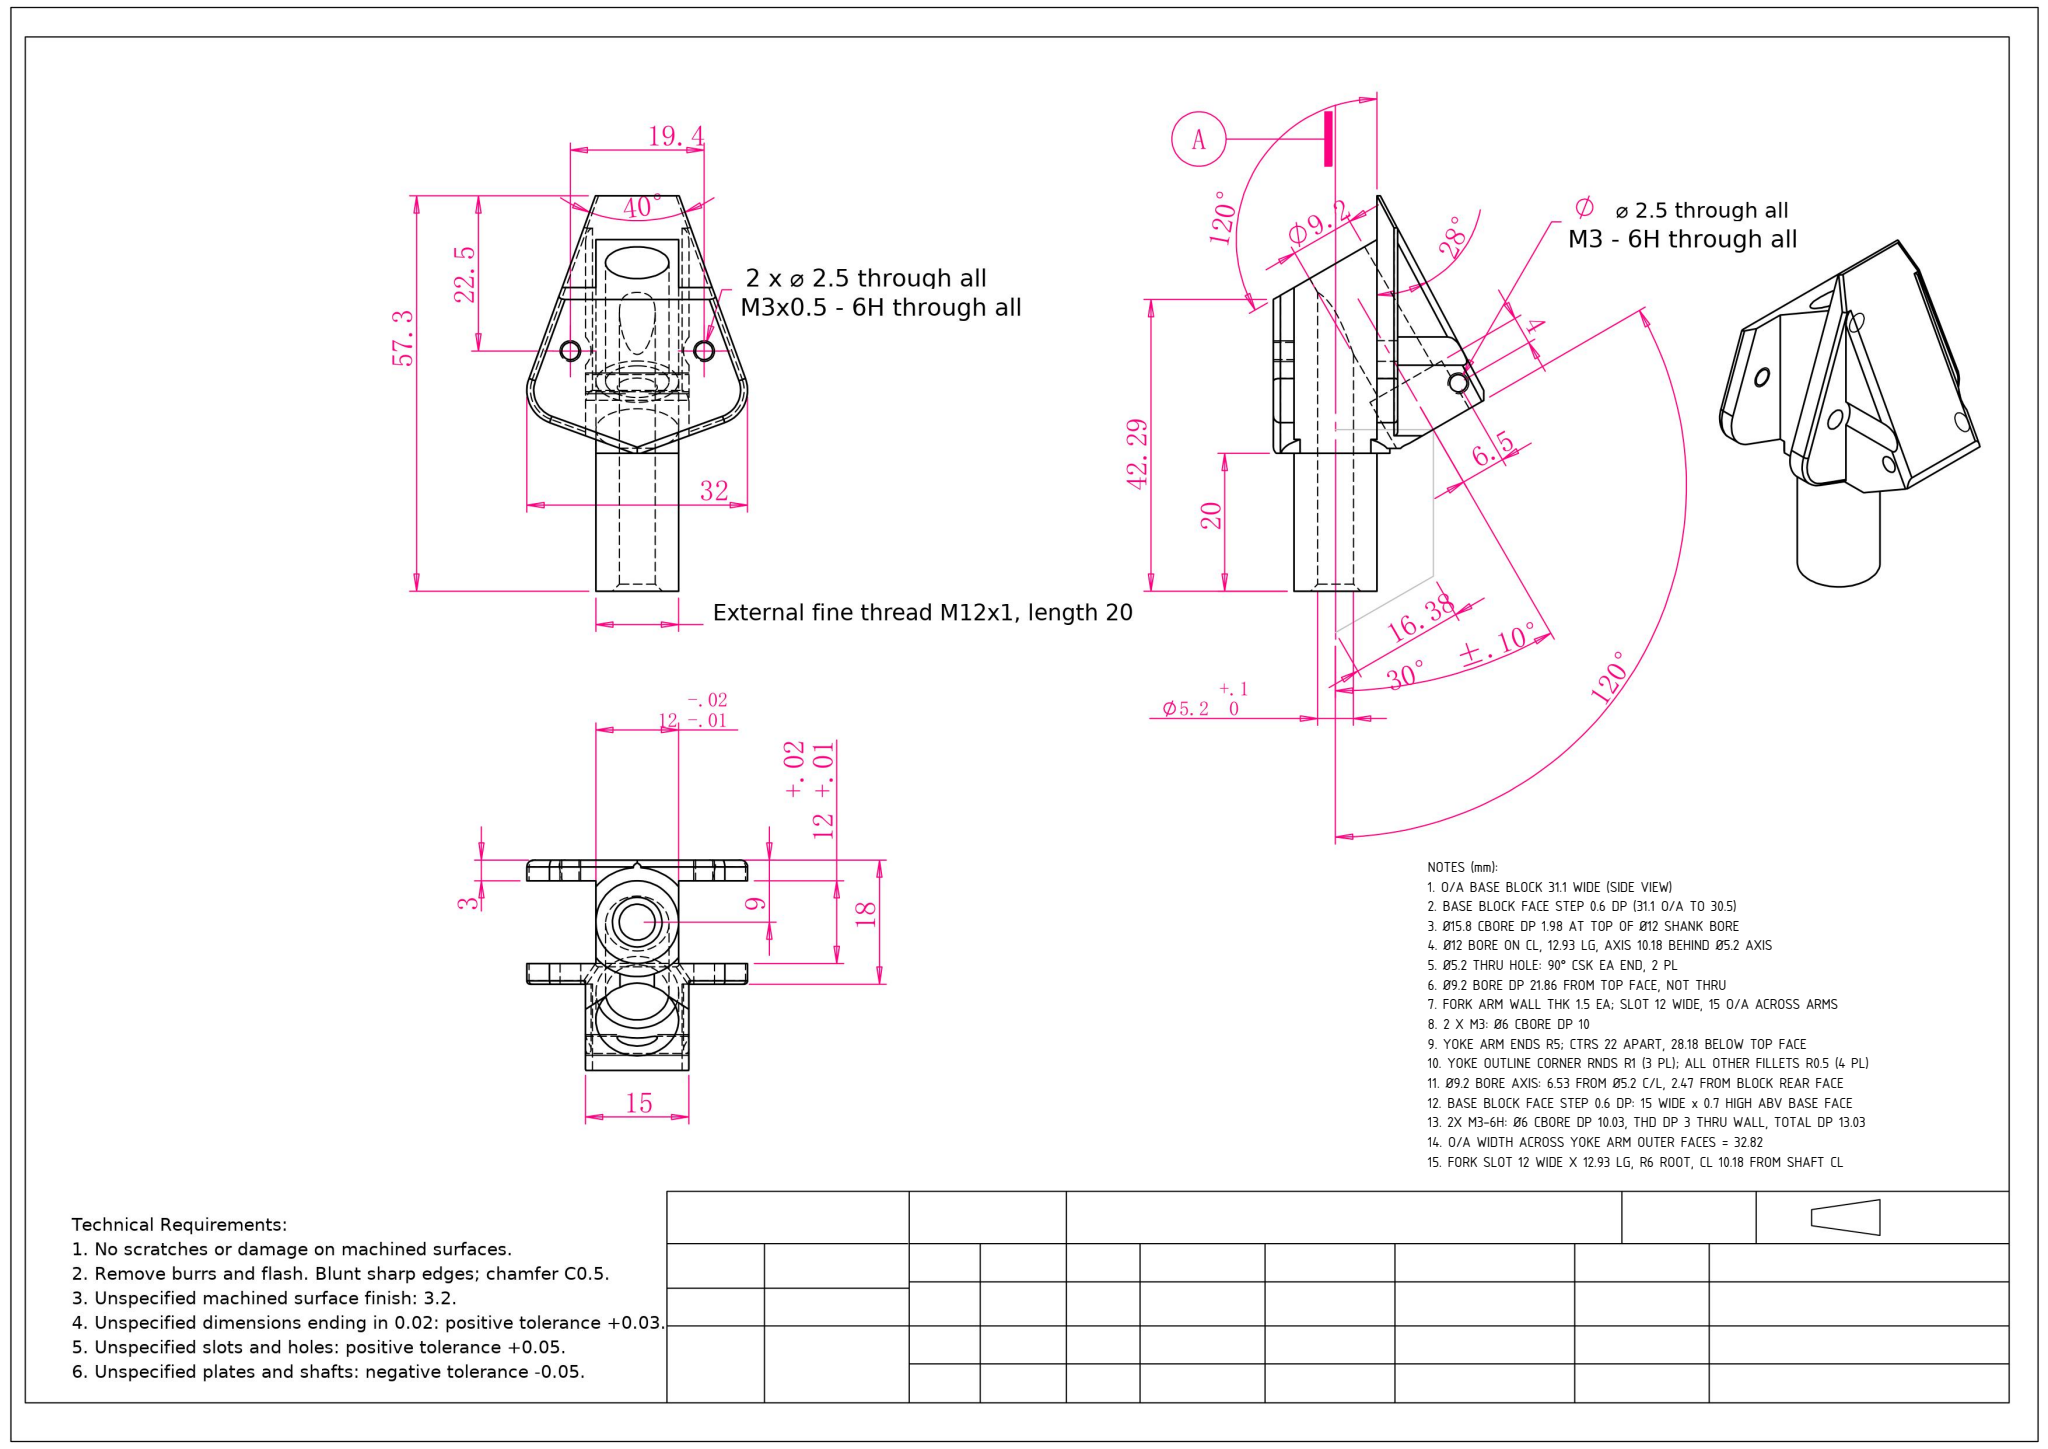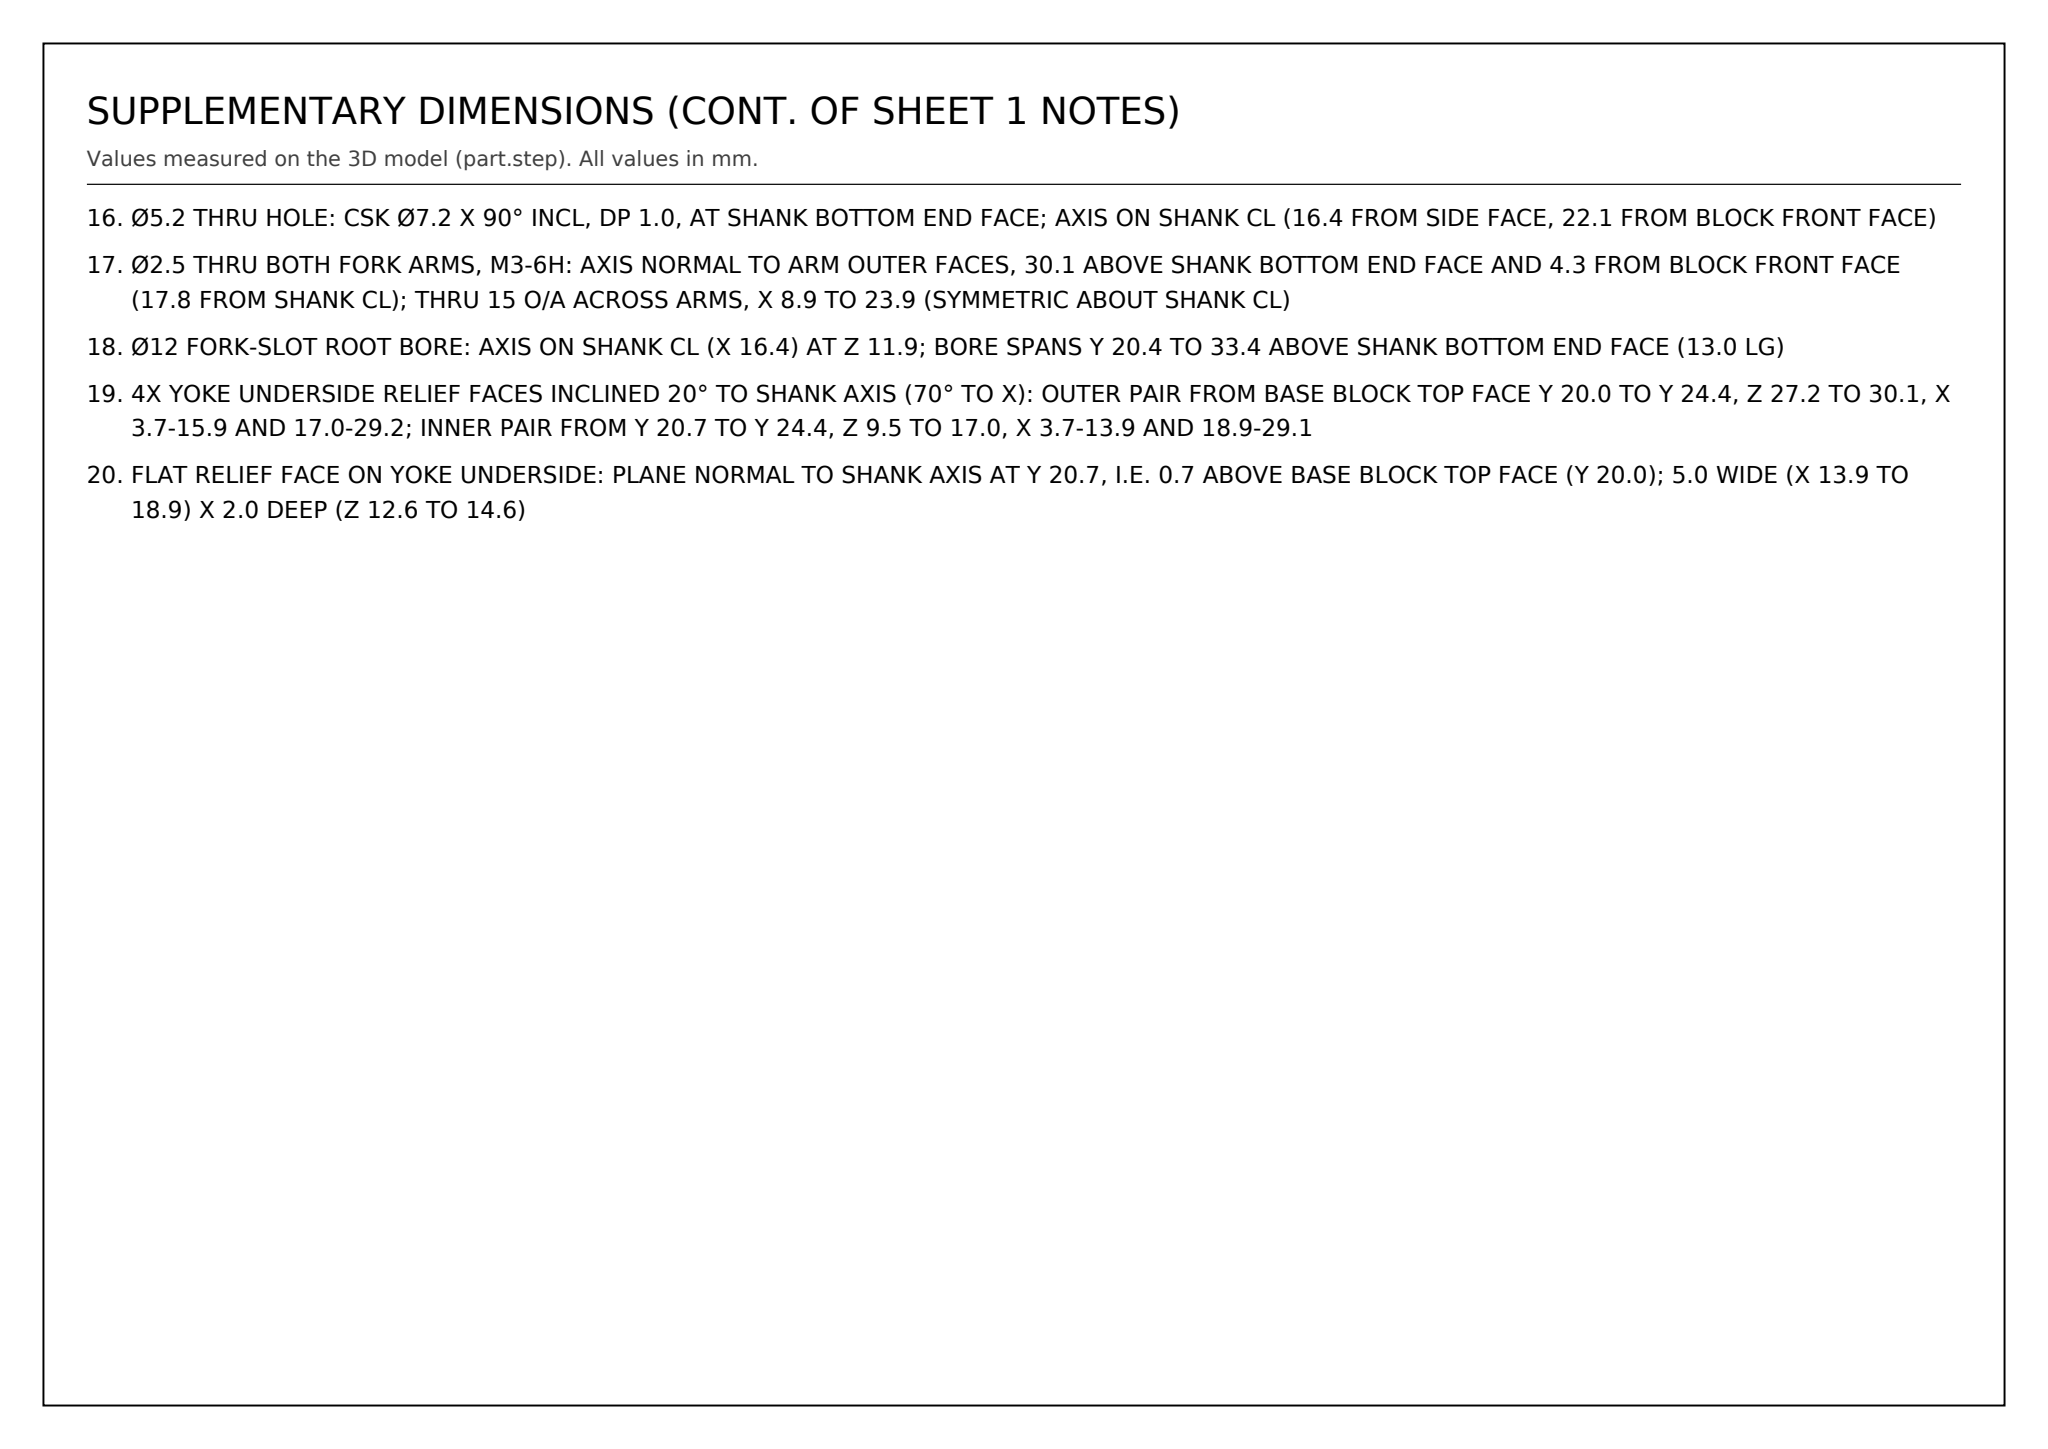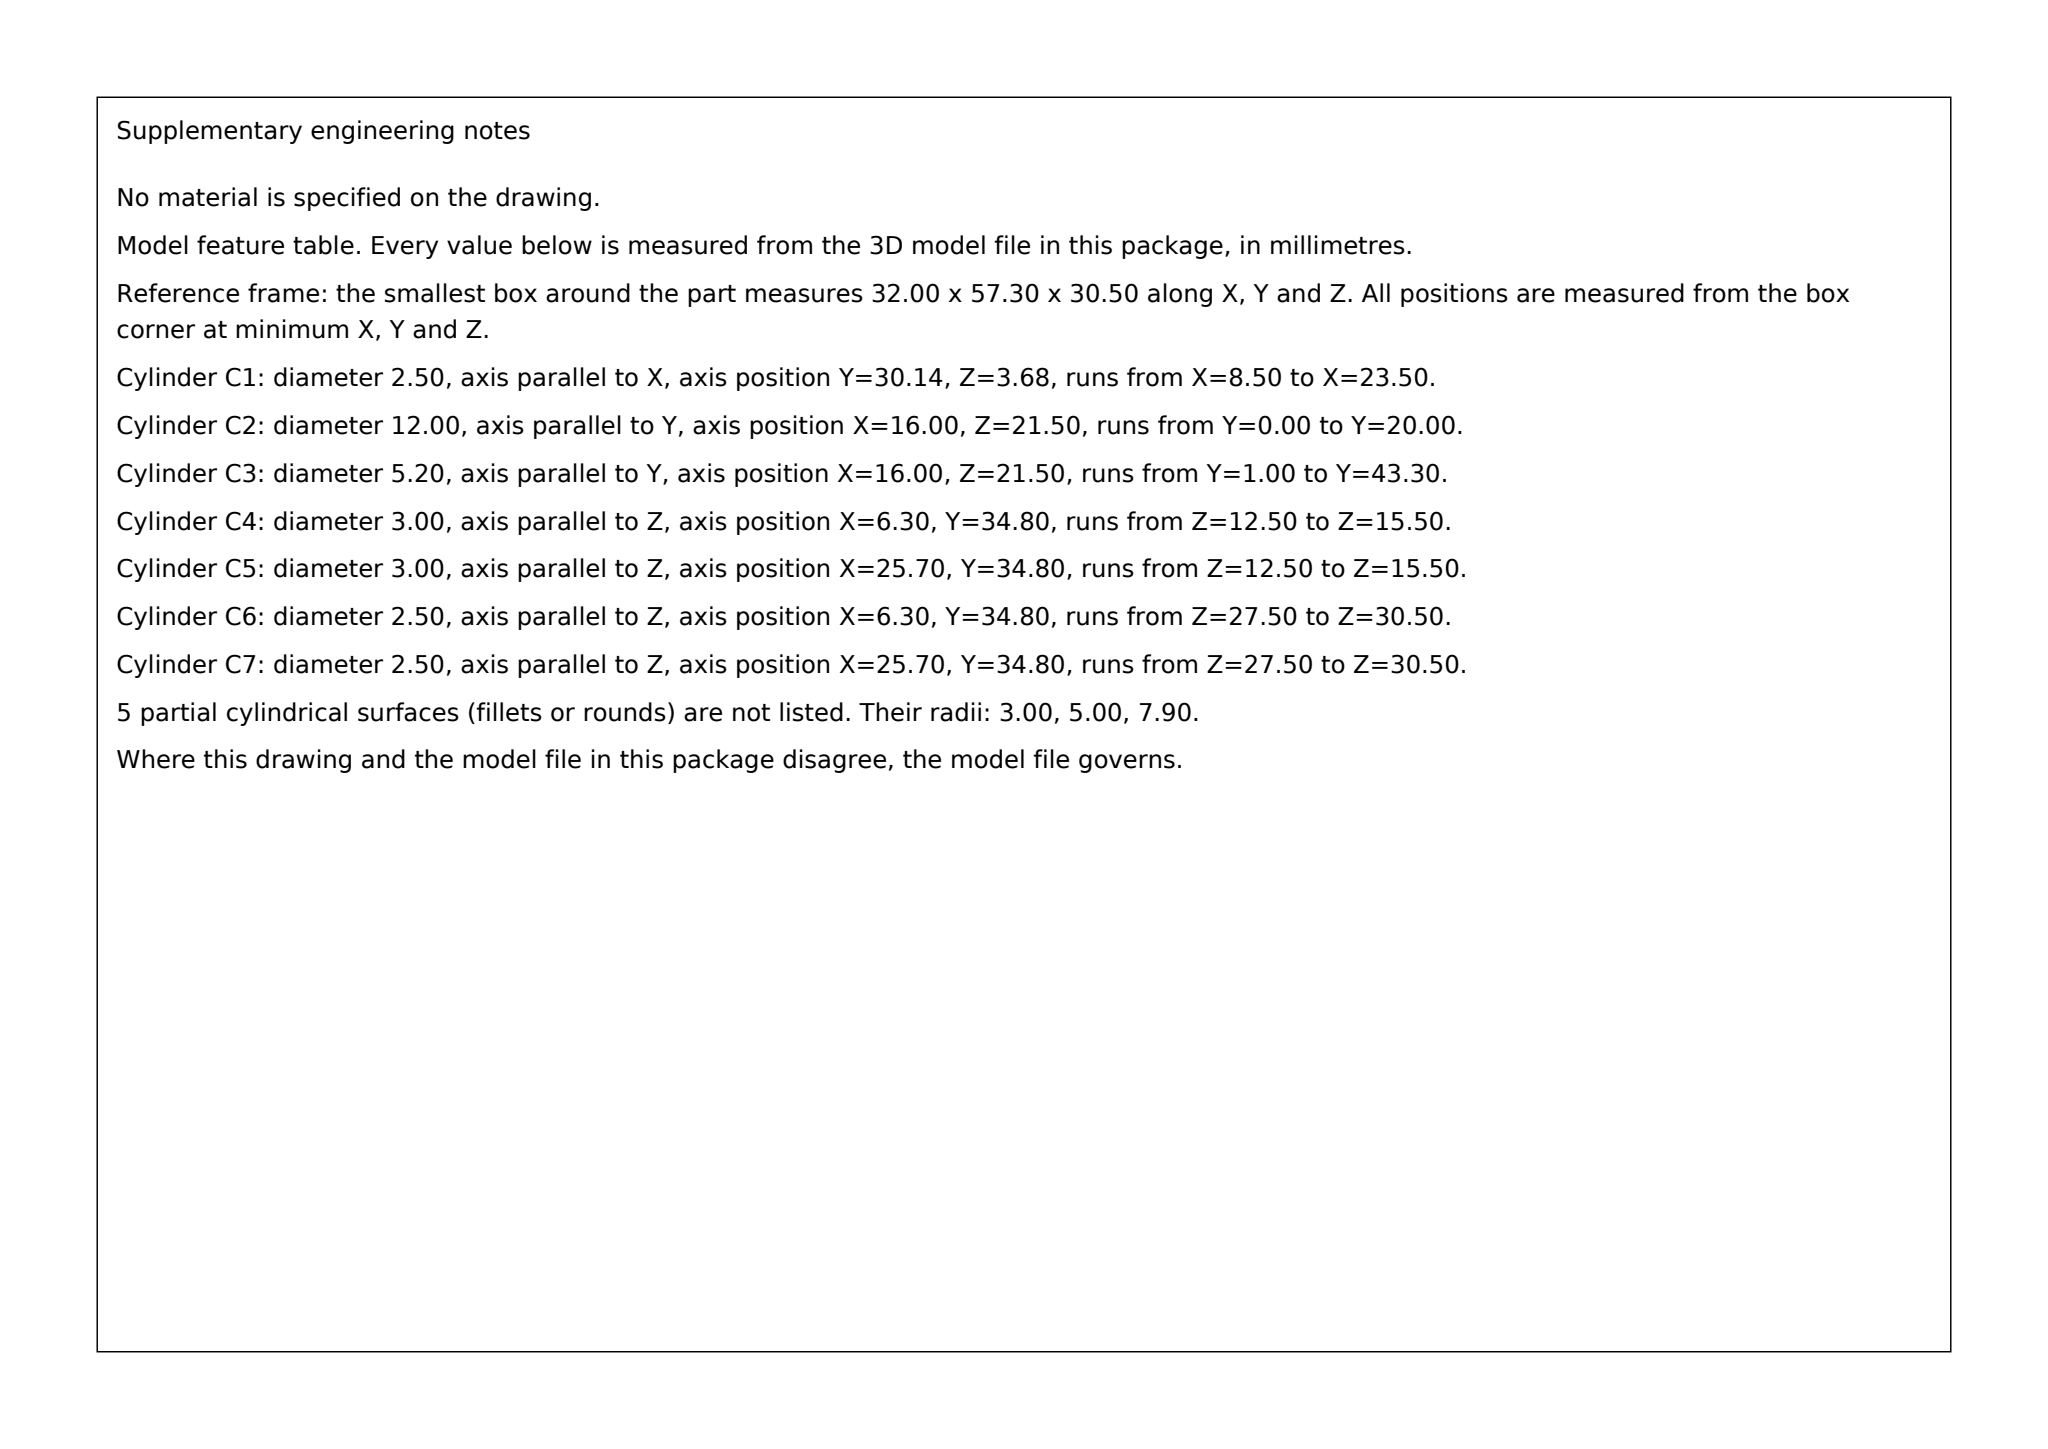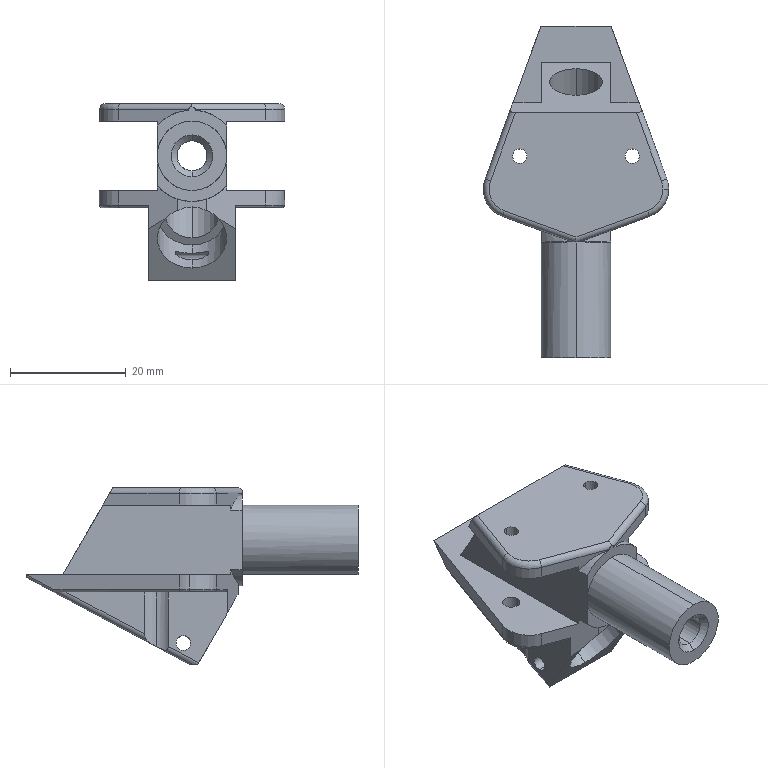Part | SolidWorks | mm | 1 solid | 82 faces | box 32 x 57.3 x 30.5 mm | volume 10257 mm3 | cylinder 43 | plane 30 | torus 7 | cone 2 | commonest cylinder face diameters 2.5 x6 10 x6 2 x6 1 x6 12 x4 3 x4 15.8 x4 6 x3
Drawing notes:
O/A BASE BLOCK 31.1 WIDE (SIDE VIEW) | from the solid: bbox_xyz z = 31.101; z planes 0.6 ... 31.1
BASE BLOCK FACE STEP 0.6 DP (31.1 O/A TO 30.5) | from the solid: z-plane at 0.6 vs bbox z 0...31.101; 31.1-0.6=30.5
Ø15.8 CBORE DP 1.98 AT TOP OF Ø12 SHANK BORE | from the solid: Ø15.8 cyl axis y at (x16.41,z22.1) L=1.98, coaxial with Ø12 (L=20) shank
Ø12 BORE ON CL, 12.93 LG, AXIS 10.18 BEHIND Ø5.2 AXIS | from the solid: cyl dia12 axis y at (x16.41,z11.92) L=12.93; 22.10-11.92=10.18; x16.41 = CL
Ø5.2 THRU HOLE: 90° CSK EA END, 2 PL | from the solid: cones [90.0, 5.2] count 2 on Ø5.2 y-axis hole (len 42.3)
Ø9.2 BORE DP 21.86 FROM TOP FACE, NOT THRU | from the solid: cyl [9.2, axis y, (16.41, 28.63), L=21.86]; top plane y=57.3 -> ends y=35.44
FORK ARM WALL THK 1.5 EA; SLOT 12 WIDE, 15 O/A ACROSS ARMS | from the solid: x planes 8.91 & 10.41, 22.41 & 23.91 -> 1.5 thk; 10.41-22.41=12; 23.91-8.91=15
2 X M3: Ø6 CBORE DP 10 | from the solid: Ø6 cyls axis z at (6.71,34.8) & (26.11,34.8), L=10.03 (9.44 cut by face)
YOKE ARM ENDS R5; CTRS 22 APART, 28.18 BELOW TOP FACE | from the solid: Ø10 cyls axis z at (5.41,29.12) & (27.41,29.12); 27.41-5.41=22; 57.3-29.12=28.18
YOKE OUTLINE CORNER RNDS R1 (3 PL); ALL OTHER FILLETS R0.5 (4 PL) | from the solid: fillet_radii: [1.0, 3] on triangular-outline corners; [0.5, 4] remaining edges
Ø9.2 BORE AXIS: 6.53 FROM Ø5.2 C/L, 2.47 FROM BLOCK REAR FACE | from the solid: Ø9.2 y-axis cyl at (x16.41,z28.63); Ø5.2 y-axis cyl at (x16.41,z22.10) -> 6.53 offset; z plane 31.1 rear face -> 2.47
BASE BLOCK FACE STEP 0.6 DP: 15 WIDE x 0.7 HIGH ABV BASE FACE | from the solid: z plane 0.6 (step face); x planes 8.91 & 23.91 -> 15 wide, symm about C/L x16.41; y planes 20.0 (base face) & 20.7 -> 0.7 high
2X M3-6H: Ø6 CBORE DP 10.03, THD DP 3 THRU WALL, TOTAL DP 13.03 | from the solid: Ø6 z-cyl at (6.71,34.8) & (26.11,34.8) L=10.03 (one split seg 9.44); Ø2.5/Ø3 z-cyl same axes L=3.0; wall planes z=28.1 to z=31.1 = 3 THK
O/A WIDTH ACROSS YOKE ARM OUTER FACES = 32.82 | from the solid: bbox_xyz x = 32.824 (vs x-planes 8.91/23.91 = 15 O/A across fork arms)
FORK SLOT 12 WIDE X 12.93 LG, R6 ROOT, CL 10.18 FROM SHAFT CL | from the solid: x-planes 10.41/22.41 = 12 slot; Ø12 y-cyl at (x16.41,z11.92) L=12.93 is slot root (R6); M12 shaft/Ø5.2 axis at z=22.1 -> 22.1-11.92=10.18
Ø5.2 THRU HOLE: CSK Ø7.2 X 90° INCL, DP 1.0, AT SHANK BOTTOM END FACE; AXIS ON SHANK CL (16.4 FROM SIDE FACE, 22.1 FROM BLOCK FRONT FACE) | from the solid: cones[90.0, ref_dia 5.2, bbox_from [12.8,0.0,18.5] / [16.4,0.0,18.5], size [3.6,1.0,7.2]] with hole/bore Ø5.2 axis y at [16.4,-,22.1] from y0.0 (1.0) to 43.3
Ø2.5 THRU BOTH FORK ARMS, M3-6H: AXIS NORMAL TO ARM OUTER FACES, 30.1 ABOVE SHANK BOTTOM END FACE AND 4.3 FROM BLOCK FRONT FACE (17.8 FROM SHANK CL); THRU 15 O/A ACROSS ARMS, X 8.9 TO 23.9 (SYMMETRIC ABOUT SHANK CL) | from the solid: cylinders hole/bore Ø2.5 axis x, axis_pos [y 30.1, z 4.3], from 8.9 to 23.9; shank Ø12 axis y at [16.4,-,22.1]
Ø12 FORK-SLOT ROOT BORE: AXIS ON SHANK CL (X 16.4) AT Z 11.9; BORE SPANS Y 20.4 TO 33.4 ABOVE SHANK BOTTOM END FACE (13.0 LG) | from the solid: cylinders: hole/bore dia 12.0 inclined, axis_pos [16.4,null,11.9], from 20.4 to 33.4
4X YOKE UNDERSIDE RELIEF FACES INCLINED 20° TO SHANK AXIS (70° TO X): OUTER PAIR FROM BASE BLOCK TOP FACE Y 20.0 TO Y 24.4, Z 27.2 TO 30.1, X 3.7-15.9 AND 17.0-29.2; INNER PAIR FROM Y 20.7 TO Y 24.4, Z 9.5 TO 17.0, X 3.7-13.9 AND 18.9-29.1 | from the solid: inclined_planes angle_to_xyz [70,20,90] x4 at bbox_from [17.0,20.0,27.2], [3.7,20.0,27.2], [18.9,20.7,9.5], [3.7,20.7,9.5]
FLAT RELIEF FACE ON YOKE UNDERSIDE: PLANE NORMAL TO SHANK AXIS AT Y 20.7, I.E. 0.7 ABOVE BASE BLOCK TOP FACE (Y 20.0); 5.0 WIDE (X 13.9 TO 18.9) X 2.0 DEEP (Z 12.6 TO 14.6) | from the solid: axis_planes: ['y',20.7, extent {'x':[13.9,18.9],'z':[12.6,14.6]}, area 6]
build123d program:
from build123d import *

# Parameters (mm, degrees)
SKETCH1_R                    = 10
EXTRUDE1_DEPTH               = 18.8
SKETCH2_R                    = 7.9
EXTRUDE2_DEPTH               = 37
EXTRUDE3_DEPTH               = 3.5
CUT_EXTRUDE1_DEPTH           = 2.5
CUT_EXTRUDE2_DEPTH           = 50
EXTRUDE5_DEPTH               = 14
CUT_EXTRUDE3_DEPTH           = 12.5
CUT_EXTRUDE4_DEPTH           = 50
CUT_EXTRUDE5_DEPTH           = 50
EXTRUDE9_DEPTH               = 0.5
CUT_EXTRUDE18_DEPTH          = 250
FILLET15_R                   = 1
FILLET16_R                   = 1
FILLET17_R                   = 1
SKETCH11_R                   = 1.2
CUT_EXTRUDE7_DEPTH           = 5
F_3_0_3_DIAMETER_HOLE1_D     = 3
F_3_0_3_DIAMETER_HOLE1_DEPTH = 8.5
SKETCH14_R                   = 2.6
CUT_EXTRUDE8_DEPTH           = 69.74
M16_TAPPED_HOLE1_D           = 14
M16_TAPPED_HOLE1_DEPTH       = 13
M16_TAPPED_HOLE1_TIP         = 4.206
EXTRUDE10_REACH              = 70.74
SKETCH52_R                   = 2.6
SKETCH52_R_2                 = 2.55
CUT_EXTRUDE9_REACH           = 60.671
SKETCH17_R                   = 4.6
SKETCH18_R                   = 6
CUT_EXTRUDE10_DEPTH          = 8
EXTRUDE8_REACH               = 70.74
SKETCH30_R                   = 7
SKETCH30_R_2                 = 2.55
SKETCH31_OUTSIDE_W           = 49.522
SKETCH31_OUTSIDE_H           = 49.022
SKETCH31_OUTSIDE_R           = 6
CUT_EXTRUDE17_DEPTH          = 26
CHAMFER1_SIZE                = 1
CUT_EXTRUDE19_DEPTH          = 71.379
CUT_EXTRUDE20_DEPTH          = 71.379
CUT_EXTRUDE21_DEPTH          = 71.379
M3_TAPPED_HOLE5_D            = 2.5
M3_TAPPED_HOLE6_D            = 2.5
SKETCH50_R                   = 3
SKETCH50_R_2                 = 3
CUT_EXTRUDE23_DEPTH          = 68.727
FILLET18_R                   = 0.5
SKETCH53_R                   = 6
CUT_EXTRUDE24_DEPTH          = 6
SKETCH54_R                   = 2.6
CUT_EXTRUDE25_DEPTH          = 64.258
CHAMFER2_SIZE                = 1


with BuildPart() as part:
    # Sketch1 → Extrude1 (new body)
    with BuildSketch(Plane(origin=(0, 0, 0), x_dir=(1, 0, 0), z_dir=(0, 1, 0))):
        with Locations(Location((0, 0, 0), (0, 0, 270))):
            Circle(SKETCH1_R)
    extrude(amount=EXTRUDE1_DEPTH)

    # Sketch2 → Extrude2 (add)
    with BuildSketch(Plane(origin=(0, 18.8, 0), x_dir=(-1, 0, 0), z_dir=(0, 1, 0))):
        with Locations(Location((0, 0, 0), (0, 0, 90))):
            Circle(SKETCH2_R)
    extrude(amount=EXTRUDE2_DEPTH)

    # Sketch3 → Extrude3 (add)
    with BuildSketch(Plane.XY.offset(8.5)):
        with BuildLine():
            Line((0, 25.8), (12.71, 30.426))
            ThreePointArc((12.71, 30.426), (15.532, 33.011), (15.698, 36.835))
            Line((15.698, 36.835), (6.066, 63.3))
            Line((6.066, 63.3), (-6.066, 63.3))
            Line((-6.066, 63.3), (-15.698, 36.835))
            ThreePointArc((-15.698, 36.835), (-15.532, 33.011), (-12.71, 30.426))
            Line((-12.71, 30.426), (0, 25.8))
        make_face()
    extrude3 = extrude(amount=-EXTRUDE3_DEPTH)

    # Mirror1: Extrude3 across plane
    add(extrude3.mirror(Plane.XY.offset(0.5)))

    # Sketch4 → Cut-Extrude1 (cut)
    with BuildSketch(Plane(origin=(8.5, 0, 0), x_dir=(0, 0, -1), z_dir=(1, 0, 0))):
        with BuildLine():
            Line((4, 36.835), (4, 63.3))
            Line((4, 63.3), (-5, 63.3))
            Line((-5, 63.3), (-5, 36.835))
            Line((-5, 36.835), (-5, 26.3))
            ThreePointArc((-5, 26.3), (-0.5, 21.8), (4, 26.3))
            Line((4, 26.3), (4, 36.835))
        make_face()
    cut_extrude1 = extrude(amount=-CUT_EXTRUDE1_DEPTH, mode=Mode.SUBTRACT)

    # Mirror2: Cut-Extrude1 across plane
    add(cut_extrude1.mirror(Plane(origin=(0, 0, 0), x_dir=(0, 0, 1), z_dir=(1, 0, 0))), mode=Mode.SUBTRACT)

    # Sketch5 → Cut-Extrude2 (cut, symmetric)
    with BuildSketch(Plane(origin=(0, 0, 0), x_dir=(0, 0, -1), z_dir=(1, 0, 0))):
        Polygon((4, 55.8), (-8.5, 48.583), (-8.5, 63.3), (4, 63.3), align=None)
    extrude(amount=CUT_EXTRUDE2_DEPTH, both=True, mode=Mode.SUBTRACT)

    # Sketch6 → Extrude5 (add)
    with BuildSketch(Plane(origin=(0, 0, -7.5), x_dir=(-1, 0, 0), z_dir=(0, 0, -1))):
        with BuildLine():
            Line((-2.482, 26.703), (2.482, 26.703))
            Line((2.482, 26.703), (12.71, 30.426))
            ThreePointArc((12.71, 30.426), (15.532, 33.011), (15.698, 36.835))
            Line((15.698, 36.835), (6.066, 63.3))
            Line((6.066, 63.3), (-6.066, 63.3))
            Line((-6.066, 63.3), (-15.698, 36.835))
            ThreePointArc((-15.698, 36.835), (-15.532, 33.011), (-12.71, 30.426))
            Line((-12.71, 30.426), (-2.482, 26.703))
        make_face()
    extrude(amount=EXTRUDE5_DEPTH)

    # Sketch7 → Cut-Extrude3 (cut)
    with BuildSketch(Plane(origin=(0, 0, -21.5), x_dir=(-1, 0, 0), z_dir=(0, 0, -1))):
        with BuildLine():
            Line((-19.5, 21.015), (-10.465, 23.436))
            ThreePointArc((-10.465, 23.436), (-8.327, 24.865), (-7.5, 27.3))
            Line((-7.5, 27.3), (-7.5, 63.3))
            Line((-7.5, 63.3), (-19.5, 63.3))
            Line((-19.5, 63.3), (-19.5, 21.015))
        make_face()
        with BuildLine():
            Line((19.5, 63.3), (19.5, 21.015))
            Line((19.5, 21.015), (10.465, 23.436))
            ThreePointArc((10.465, 23.436), (8.327, 24.865), (7.5, 27.3))
            Line((7.5, 27.3), (7.5, 63.3))
            Line((7.5, 63.3), (19.5, 63.3))
        make_face()
    extrude(amount=-CUT_EXTRUDE3_DEPTH, mode=Mode.SUBTRACT)

    # Sketch8 → Cut-Extrude4 (cut, symmetric)
    with BuildSketch(Plane(origin=(0, 0, 0), x_dir=(0, 0, -1), z_dir=(1, 0, 0))):
        Polygon((7.9, 25.8), (21.5, 33.652), (21.5, 25.8), align=None)
    extrude(amount=CUT_EXTRUDE4_DEPTH, both=True, mode=Mode.SUBTRACT)

    # Sketch9 → Cut-Extrude5 (cut, symmetric)
    with BuildSketch(Plane(origin=(0, 0, 0), x_dir=(0, 0, -1), z_dir=(1, 0, 0))):
        Polygon((6.5, 63.3), (21.5, 35.089), (21.5, 63.3), align=None)
    extrude(amount=CUT_EXTRUDE5_DEPTH, both=True, mode=Mode.SUBTRACT)

    # Sketch32 → Extrude9 (add)
    with BuildSketch(Plane.XY.offset(8.5)):
        with BuildLine():
            Line((0, 25.8), (12.71, 30.426))
            ThreePointArc((12.71, 30.426), (15.532, 33.011), (15.698, 36.835))
            Line((15.698, 36.835), (11.422, 48.583))
            Line((11.422, 48.583), (-11.422, 48.583))
            Line((-11.422, 48.583), (-15.698, 36.835))
            ThreePointArc((-15.698, 36.835), (-15.532, 33.011), (-12.71, 30.426))
            Line((-12.71, 30.426), (0, 25.8))
        make_face()
    extrude(amount=EXTRUDE9_DEPTH)

    # Sketch34 → Cut-Extrude18 (cut, symmetric)
    with BuildSketch(Plane.ZY.offset(6)):
        Polygon((5, 50.604), (9, 48.294), (9.125, 48.511), (5.125, 50.82), align=None)
    extrude(amount=CUT_EXTRUDE18_DEPTH, both=True, mode=Mode.SUBTRACT)

    # Fillet15
    fillet15_edges = [part.edges().sort_by_distance(p)[0] for p in [
        (-7.5, 46.844, -15.25),
    ]]
    fillet(fillet15_edges, radius=FILLET15_R)

    # Fillet16
    fillet16_edges = [part.edges().sort_by_distance(p)[0] for p in [
        (7.5, 46.844, -15.25),
    ]]
    fillet(fillet16_edges, radius=FILLET16_R)

    # Fillet17
    fillet17_edges = [part.edges().sort_by_distance(p)[0] for p in [
        (-15.532, 33.011, 9),
        (-6.355, 28.113, 9),
        (6.355, 28.113, 9),
        (15.532, 33.011, 9),
        (13.613, 42.565, 9),
        (-13.613, 42.565, 9),
    ]]
    fillet(fillet17_edges, radius=FILLET17_R)

    # Sketch11 → Cut-Extrude7 (cut)
    with BuildSketch(Plane.XY.offset(9)):
        with Locations((-9.7, 40.8)):
            Circle(SKETCH11_R)
        with Locations((9.7, 40.8)):
            Circle(SKETCH11_R)
    extrude(amount=-CUT_EXTRUDE7_DEPTH, mode=Mode.SUBTRACT)

    # 3.0 _3_ Diameter Hole1
    with Locations(Plane.XY.offset(-4)):
        with Locations((-9.7, 40.8), (9.7, 40.8)):
            Hole(F_3_0_3_DIAMETER_HOLE1_D / 2, depth=F_3_0_3_DIAMETER_HOLE1_DEPTH)

    # Sketch14 → Cut-Extrude8 (cut, through all)
    with BuildSketch(Plane.XZ):
        with Locations(Location((0, 0, 0), (0, 0, 270))):
            Circle(SKETCH14_R)
    extrude(amount=-CUT_EXTRUDE8_DEPTH, mode=Mode.SUBTRACT)

    # M16 Tapped Hole1
    with Locations(Plane.XZ):
        with Locations((0, 0)):
            Hole(M16_TAPPED_HOLE1_D / 2, depth=M16_TAPPED_HOLE1_DEPTH)
            with Locations((0, 0, -(M16_TAPPED_HOLE1_DEPTH + M16_TAPPED_HOLE1_TIP / 2))):  # 118° drill point
                Cone(0, M16_TAPPED_HOLE1_D / 2, M16_TAPPED_HOLE1_TIP, mode=Mode.SUBTRACT)

    # Extrude10: up to this plane
    extrude10_end = Plane(origin=(-50, 55.8, -4), z_dir=(0, -0.866, -0.5))
    # Sketch52 → Extrude10 (add, up to the surface)
    with BuildSketch(Plane.XZ, mode=Mode.PRIVATE) as extrude10_sk1:
        with Locations(Location((0, 0, 0), (0, 0, 270))):
            Circle(SKETCH52_R)
        with Locations(Location((0, 0, 0), (0, 0, 270))):
            Circle(SKETCH52_R_2, mode=Mode.SUBTRACT)
    extrude10_tool1 = split(extrude(extrude10_sk1.sketch, amount=-EXTRUDE10_REACH, mode=Mode.PRIVATE), bisect_by=extrude10_end, keep=Keep.BOTH, mode=Mode.PRIVATE)
    add(extrude10_tool1.solids().sort_by_distance((0, 0, 2.593))[0])

    # Sketch17 → Cut-Extrude9 (cut, up to next)
    with BuildSketch(Plane(origin=(0, 15.929, 9.197), x_dir=(1, 0, 0), z_dir=(0, -0.866, -0.5)), mode=Mode.PRIVATE) as cut_extrude9_sk1:
        with Locations(Location((0, -27, 0), (0, 0, 270))):
            Circle(SKETCH17_R)
    cut_extrude9_tool1 = extrude(cut_extrude9_sk1.sketch, amount=-CUT_EXTRUDE9_REACH, mode=Mode.PRIVATE) & part.part
    add(cut_extrude9_tool1.solids().sort_by_distance((0, 29.429, -14.186))[0], mode=Mode.SUBTRACT)

    # Sketch18 → Cut-Extrude10 (cut, symmetric)
    with BuildSketch(Plane(origin=(0, 15.929, 9.197), x_dir=(1, 0, 0), z_dir=(0, -0.866, -0.5))):
        with Locations(Location((0, -27, 0), (0, 0, 270))):
            Circle(SKETCH18_R)
    extrude(amount=CUT_EXTRUDE10_DEPTH, both=True, mode=Mode.SUBTRACT)

    # Sketch30 → Extrude8 (add, up to next)
    with BuildSketch(Plane.XZ, mode=Mode.PRIVATE) as extrude8_sk1:
        Circle(SKETCH30_R)
        with Locations(Location((0, 0, 0), (0, 0, 270))):
            Circle(SKETCH30_R_2, mode=Mode.SUBTRACT)
    extrude8_tool1 = extrude(extrude8_sk1.sketch, amount=-EXTRUDE8_REACH, mode=Mode.PRIVATE) - part.part
    add(extrude8_tool1.solids().sort_by_distance((-6.802, 0, 0))[0])

    # Sketch31 outside → Cut-Extrude17 (cut)
    with BuildSketch(Plane.XZ):
        with Locations((0, -5.75)):
            Rectangle(SKETCH31_OUTSIDE_W, SKETCH31_OUTSIDE_H)
        with Locations(Location((0, 0, 0), (0, 0, 270))):
            Circle(SKETCH31_OUTSIDE_R, mode=Mode.SUBTRACT)
    extrude(amount=-CUT_EXTRUDE17_DEPTH, mode=Mode.SUBTRACT)

    # Chamfer1
    chamfer1_edges = [part.edges().sort_by_distance(p)[0] for p in [
        (0, 0, 2.55),
    ]]
    chamfer(chamfer1_edges, length=CHAMFER1_SIZE)

    # Sketch37 → Cut-Extrude19 (cut, through all)
    with BuildSketch(Plane(origin=(6, 0, 0), x_dir=(0, 0, -1), z_dir=(1, 0, 0))):
        with BuildLine():
            Line((-6, 63.3), (-6, 21.3))
            ThreePointArc((-6, 21.3), (0, 15.3), (6, 21.3))
            Line((6, 21.3), (6, 63.3))
            Line((6, 63.3), (-6, 63.3))
        make_face()
    extrude(amount=CUT_EXTRUDE19_DEPTH, mode=Mode.SUBTRACT)

    # Sketch38 → Cut-Extrude20 (cut, through all)
    with BuildSketch(Plane.ZY.offset(6)):
        with BuildLine():
            Line((6, 21.3), (6, 63.3))
            Line((6, 63.3), (-6, 63.3))
            Line((-6, 63.3), (-6, 21.3))
            ThreePointArc((-6, 21.3), (0, 15.3), (6, 21.3))
        make_face()
    extrude(amount=CUT_EXTRUDE20_DEPTH, mode=Mode.SUBTRACT)

    # Sketch39 → Cut-Extrude21 (cut, through all)
    with BuildSketch(Plane(origin=(6, 0, 0), x_dir=(0, 0, -1), z_dir=(1, 0, 0))):
        Polygon((4, 55.8), (6, 56.955), (6, 63.3), (4, 63.3), align=None)
    extrude(amount=-CUT_EXTRUDE21_DEPTH, mode=Mode.SUBTRACT)

    # M3 Tapped Hole5 (through all)
    with Locations(Plane.ZY.offset(7.5)):
        with Locations((-17.815, 36.143)):
            Hole(M3_TAPPED_HOLE5_D / 2)

    # M3 Tapped Hole6 (through all)
    with Locations(Plane(origin=(0, 0, 6), x_dir=(-1, 0, 0), z_dir=(0, 0, -1))):
        with Locations((-9.7, 40.8), (9.7, 40.8)):
            Hole(M3_TAPPED_HOLE6_D / 2)

    # Sketch50 → Cut-Extrude23 (cut, through all)
    with BuildSketch(Plane(origin=(0, 0, -9), x_dir=(-1, 0, 0), z_dir=(0, 0, -1))):
        with Locations((-9.7, 40.8)):
            Circle(SKETCH50_R)
        with Locations((9.7, 40.8)):
            Circle(SKETCH50_R_2)
    extrude(amount=CUT_EXTRUDE23_DEPTH, mode=Mode.SUBTRACT)

    # Fillet18
    fillet18_edges = [part.edges().sort_by_distance(p)[0] for p in [
        (11.738, 47.716, -9),
        (10.105, 29.478, -9),
        (15.532, 33.011, -9),
        (-15.532, 33.011, -9),
        (-10.105, 29.478, -9),
        (-11.738, 47.716, -9),
        (6.922, 60.949, -7.75),
        (-6.922, 60.949, -7.75),
    ]]
    fillet(fillet18_edges, radius=FILLET18_R)

    # Sketch53 → Cut-Extrude24 (cut)
    with BuildSketch(Plane.XZ):
        with Locations(Location((0, 0, 0), (0, 0, 270))):
            Circle(SKETCH53_R)
    extrude(amount=-CUT_EXTRUDE24_DEPTH, mode=Mode.SUBTRACT)

    # Sketch54 → Cut-Extrude25 (cut, through all)
    with BuildSketch(Plane.XZ.offset(-6)):
        with Locations(Location((0, 0, 0), (0, 0, 270))):
            Circle(SKETCH54_R)
    extrude(amount=-CUT_EXTRUDE25_DEPTH, mode=Mode.SUBTRACT)

    # Chamfer2
    chamfer2_edges = [part.edges().sort_by_distance(p)[0] for p in [
        (0, 6, 2.6),
    ]]
    chamfer(chamfer2_edges, length=CHAMFER2_SIZE)


solid = part.part